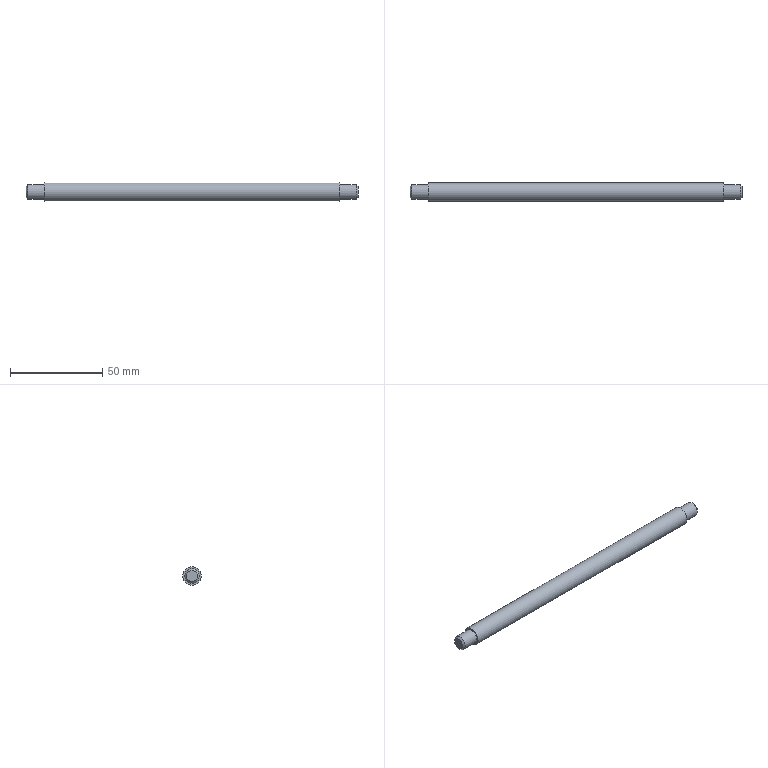Component | NX | HANDLE | 1 solid | 9 faces | box 180 x 10 x 10 mm | volume 13549 mm3 | plane 4 | cylinder 3 | cone 2 | commonest cylinder face diameters 8 x2 10 x1
STEP:
#1=CARTESIAN_POINT('',(0.,0.,0.));
#2=DIRECTION('',(0.,0.,1.));
#3=DIRECTION('',(1.,0.,0.));
#4=AXIS2_PLACEMENT_3D('',#1,#2,#3);
#5=CARTESIAN_POINT('',(80.,-135.,-189.));
#6=VERTEX_POINT('',#5);
#7=CARTESIAN_POINT('',(80.,-140.,-189.));
#8=DIRECTION('',(1.,0.,0.));
#9=DIRECTION('',(0.,1.,0.));
#10=AXIS2_PLACEMENT_3D('',#7,#8,#9);
#11=CIRCLE('',#10,5.);
#12=CARTESIAN_POINT('',(80.,-140.,-189.));
#13=DIRECTION('',(-1.,0.,0.));
#14=DIRECTION('',(0.,0.,1.));
#15=AXIS2_PLACEMENT_3D('',#12,#13,#14);
#16=CYLINDRICAL_SURFACE('',#15,5.);
#17=CARTESIAN_POINT('',(7.854,0.));
#18=DIRECTION('',(-1.,0.));
#19=VECTOR('',#18,1.);
#20=LINE('',#17,#19);
#21=(GEOMETRIC_REPRESENTATION_CONTEXT(2)PARAMETRIC_REPRESENTATION_CONTEXT()REPRESENTATION_CONTEXT('',''));
#22=DEFINITIONAL_REPRESENTATION('',(#20),#21);
#23=PCURVE('',#16,#22);
#24=CARTESIAN_POINT('',(80.,-140.,-189.));
#25=DIRECTION('',(1.,0.,0.));
#26=DIRECTION('',(0.,0.,-1.));
#27=AXIS2_PLACEMENT_3D('',#24,#25,#26);
#28=PLANE('',#27);
#29=CARTESIAN_POINT('',(0.,0.));
#30=DIRECTION('',(0.,1.));
#31=AXIS2_PLACEMENT_2D('',#29,#30);
#32=CIRCLE('',#31,5.);
#33=(GEOMETRIC_REPRESENTATION_CONTEXT(2)PARAMETRIC_REPRESENTATION_CONTEXT()REPRESENTATION_CONTEXT('',''));
#34=DEFINITIONAL_REPRESENTATION('',(#32),#33);
#35=PCURVE('',#28,#34);
#36=SURFACE_CURVE('',#11,(#23,#35),.PCURVE_S1.);
#37=EDGE_CURVE('',#6,#6,#36,.T.);
#38=ORIENTED_EDGE('',*,*,#37,.F.);
#39=CARTESIAN_POINT('',(-80.,-135.,-189.));
#40=VERTEX_POINT('',#39);
#41=CARTESIAN_POINT('',(80.,-135.,-189.));
#42=CARTESIAN_POINT('',(-80.,-135.,-189.));
#43=B_SPLINE_CURVE_WITH_KNOTS('',1,(#41,#42),.UNSPECIFIED.,.F.,.F.,(2,2),(0.,160.),.PIECEWISE_BEZIER_KNOTS.);
#44=CARTESIAN_POINT('',(7.854,0.));
#45=DIRECTION('',(0.,1.));
#46=VECTOR('',#45,1.);
#47=LINE('',#44,#46);
#48=(GEOMETRIC_REPRESENTATION_CONTEXT(2)PARAMETRIC_REPRESENTATION_CONTEXT()REPRESENTATION_CONTEXT('',''));
#49=DEFINITIONAL_REPRESENTATION('',(#47),#48);
#50=PCURVE('',#16,#49);
#51=CARTESIAN_POINT('',(1.571,0.));
#52=DIRECTION('',(0.,1.));
#53=VECTOR('',#52,1.);
#54=LINE('',#51,#53);
#55=(GEOMETRIC_REPRESENTATION_CONTEXT(2)PARAMETRIC_REPRESENTATION_CONTEXT()REPRESENTATION_CONTEXT('',''));
#56=DEFINITIONAL_REPRESENTATION('',(#54),#55);
#57=PCURVE('',#16,#56);
#58=SEAM_CURVE('',#43,(#50,#57),.PCURVE_S1.);
#59=EDGE_CURVE('',#6,#40,#58,.T.);
#60=ORIENTED_EDGE('',*,*,#59,.T.);
#61=CARTESIAN_POINT('',(-80.,-140.,-189.));
#62=DIRECTION('',(1.,0.,0.));
#63=DIRECTION('',(0.,1.,0.));
#64=AXIS2_PLACEMENT_3D('',#61,#62,#63);
#65=CIRCLE('',#64,5.);
#66=CARTESIAN_POINT('',(7.854,160.));
#67=DIRECTION('',(-1.,0.));
#68=VECTOR('',#67,1.);
#69=LINE('',#66,#68);
#70=(GEOMETRIC_REPRESENTATION_CONTEXT(2)PARAMETRIC_REPRESENTATION_CONTEXT()REPRESENTATION_CONTEXT('',''));
#71=DEFINITIONAL_REPRESENTATION('',(#69),#70);
#72=PCURVE('',#16,#71);
#73=CARTESIAN_POINT('',(-80.,-140.,-189.));
#74=DIRECTION('',(1.,0.,0.));
#75=DIRECTION('',(0.,0.,-1.));
#76=AXIS2_PLACEMENT_3D('',#73,#74,#75);
#77=PLANE('',#76);
#78=CARTESIAN_POINT('',(0.,0.));
#79=DIRECTION('',(0.,1.));
#80=AXIS2_PLACEMENT_2D('',#78,#79);
#81=CIRCLE('',#80,5.);
#82=(GEOMETRIC_REPRESENTATION_CONTEXT(2)PARAMETRIC_REPRESENTATION_CONTEXT()REPRESENTATION_CONTEXT('',''));
#83=DEFINITIONAL_REPRESENTATION('',(#81),#82);
#84=PCURVE('',#77,#83);
#85=SURFACE_CURVE('',#65,(#72,#84),.PCURVE_S1.);
#86=EDGE_CURVE('',#40,#40,#85,.T.);
#87=ORIENTED_EDGE('',*,*,#86,.T.);
#88=ORIENTED_EDGE('',*,*,#59,.F.);
#89=EDGE_LOOP('',(#38,#60,#87,#88));
#90=FACE_BOUND('',#89,.T.);
#91=ADVANCED_FACE('',(#90),#16,.T.);
#92=CARTESIAN_POINT('',(80.,-140.,-193.));
#93=VERTEX_POINT('',#92);
#94=CARTESIAN_POINT('',(80.,-140.,-189.));
#95=DIRECTION('',(-1.,0.,0.));
#96=DIRECTION('',(0.,0.,-1.));
#97=AXIS2_PLACEMENT_3D('',#94,#95,#96);
#98=CIRCLE('',#97,4.);
#99=CARTESIAN_POINT('',(4.,0.));
#100=CARTESIAN_POINT('',(4.,-6.928));
#101=CARTESIAN_POINT('',(-2.,-3.464));
#102=CARTESIAN_POINT('',(-8.,-0.));
#103=CARTESIAN_POINT('',(-2.,3.464));
#104=CARTESIAN_POINT('',(4.,6.928));
#105=CARTESIAN_POINT('',(4.,0.));
#106=(BOUNDED_CURVE()B_SPLINE_CURVE(2,(#99,#100,#101,#102,#103,#104,#105),.UNSPECIFIED.,.T.,.F.)B_SPLINE_CURVE_WITH_KNOTS((1,2,2,2,2,1),(-2.094,0.,2.094,4.189,6.283,8.378),.UNSPECIFIED.)CURVE()GEOMETRIC_REPRESENTATION_ITEM()RATIONAL_B_SPLINE_CURVE((1.,0.5,1.,0.5,1.,0.5,1.))REPRESENTATION_ITEM(''));
#107=(GEOMETRIC_REPRESENTATION_CONTEXT(2)PARAMETRIC_REPRESENTATION_CONTEXT()REPRESENTATION_CONTEXT('',''));
#108=DEFINITIONAL_REPRESENTATION('',(#106),#107);
#109=PCURVE('',#28,#108);
#110=CARTESIAN_POINT('',(90.,-140.,-189.));
#111=DIRECTION('',(-1.,0.,0.));
#112=DIRECTION('',(0.,0.,1.));
#113=AXIS2_PLACEMENT_3D('',#110,#111,#112);
#114=CYLINDRICAL_SURFACE('',#113,4.);
#115=CARTESIAN_POINT('',(3.142,10.));
#116=DIRECTION('',(1.,0.));
#117=VECTOR('',#116,1.);
#118=LINE('',#115,#117);
#119=(GEOMETRIC_REPRESENTATION_CONTEXT(2)PARAMETRIC_REPRESENTATION_CONTEXT()REPRESENTATION_CONTEXT('',''));
#120=DEFINITIONAL_REPRESENTATION('',(#118),#119);
#121=PCURVE('',#114,#120);
#122=SURFACE_CURVE('',#98,(#109,#121),.PCURVE_S1.);
#123=EDGE_CURVE('',#93,#93,#122,.T.);
#124=ORIENTED_EDGE('',*,*,#123,.T.);
#125=EDGE_LOOP('',(#124));
#126=FACE_BOUND('',#125,.T.);
#127=ORIENTED_EDGE('',*,*,#37,.T.);
#128=EDGE_LOOP('',(#127));
#129=FACE_BOUND('',#128,.T.);
#130=ADVANCED_FACE('',(#126,#129),#28,.T.);
#131=CARTESIAN_POINT('',(-80.,-140.,-193.));
#132=VERTEX_POINT('',#131);
#133=CARTESIAN_POINT('',(-80.,-140.,-189.));
#134=DIRECTION('',(-1.,0.,0.));
#135=DIRECTION('',(0.,0.,-1.));
#136=AXIS2_PLACEMENT_3D('',#133,#134,#135);
#137=CIRCLE('',#136,4.);
#138=CARTESIAN_POINT('',(4.,0.));
#139=CARTESIAN_POINT('',(4.,-6.928));
#140=CARTESIAN_POINT('',(-2.,-3.464));
#141=CARTESIAN_POINT('',(-8.,-0.));
#142=CARTESIAN_POINT('',(-2.,3.464));
#143=CARTESIAN_POINT('',(4.,6.928));
#144=CARTESIAN_POINT('',(4.,0.));
#145=(BOUNDED_CURVE()B_SPLINE_CURVE(2,(#138,#139,#140,#141,#142,#143,#144),.UNSPECIFIED.,.T.,.F.)B_SPLINE_CURVE_WITH_KNOTS((1,2,2,2,2,1),(-2.094,0.,2.094,4.189,6.283,8.378),.UNSPECIFIED.)CURVE()GEOMETRIC_REPRESENTATION_ITEM()RATIONAL_B_SPLINE_CURVE((1.,0.5,1.,0.5,1.,0.5,1.))REPRESENTATION_ITEM(''));
#146=(GEOMETRIC_REPRESENTATION_CONTEXT(2)PARAMETRIC_REPRESENTATION_CONTEXT()REPRESENTATION_CONTEXT('',''));
#147=DEFINITIONAL_REPRESENTATION('',(#145),#146);
#148=PCURVE('',#77,#147);
#149=CARTESIAN_POINT('',(90.,-140.,-189.));
#150=DIRECTION('',(-1.,0.,0.));
#151=DIRECTION('',(0.,0.,1.));
#152=AXIS2_PLACEMENT_3D('',#149,#150,#151);
#153=CYLINDRICAL_SURFACE('',#152,4.);
#154=CARTESIAN_POINT('',(3.142,170.));
#155=DIRECTION('',(1.,0.));
#156=VECTOR('',#155,1.);
#157=LINE('',#154,#156);
#158=(GEOMETRIC_REPRESENTATION_CONTEXT(2)PARAMETRIC_REPRESENTATION_CONTEXT()REPRESENTATION_CONTEXT('',''));
#159=DEFINITIONAL_REPRESENTATION('',(#157),#158);
#160=PCURVE('',#153,#159);
#161=SURFACE_CURVE('',#137,(#148,#160),.PCURVE_S1.);
#162=EDGE_CURVE('',#132,#132,#161,.T.);
#163=ORIENTED_EDGE('',*,*,#162,.F.);
#164=EDGE_LOOP('',(#163));
#165=FACE_BOUND('',#164,.T.);
#166=ORIENTED_EDGE('',*,*,#86,.F.);
#167=EDGE_LOOP('',(#166));
#168=FACE_BOUND('',#167,.T.);
#169=ADVANCED_FACE('',(#165,#168),#77,.F.);
#170=CARTESIAN_POINT('',(-90.,-140.,-192.));
#171=VERTEX_POINT('',#170);
#172=CARTESIAN_POINT('',(-90.,-140.,-189.));
#173=DIRECTION('',(-1.,0.,0.));
#174=DIRECTION('',(0.,0.,-1.));
#175=AXIS2_PLACEMENT_3D('',#172,#173,#174);
#176=CIRCLE('',#175,3.);
#177=CARTESIAN_POINT('',(-90.,-140.,-189.));
#178=DIRECTION('',(1.,0.,0.));
#179=DIRECTION('',(0.,0.,-1.));
#180=AXIS2_PLACEMENT_3D('',#177,#178,#179);
#181=PLANE('',#180);
#182=CARTESIAN_POINT('',(3.,0.));
#183=CARTESIAN_POINT('',(3.,-5.196));
#184=CARTESIAN_POINT('',(-1.5,-2.598));
#185=CARTESIAN_POINT('',(-6.,-0.));
#186=CARTESIAN_POINT('',(-1.5,2.598));
#187=CARTESIAN_POINT('',(3.,5.196));
#188=CARTESIAN_POINT('',(3.,0.));
#189=(BOUNDED_CURVE()B_SPLINE_CURVE(2,(#182,#183,#184,#185,#186,#187,#188),.UNSPECIFIED.,.T.,.F.)B_SPLINE_CURVE_WITH_KNOTS((1,2,2,2,2,1),(-2.094,0.,2.094,4.189,6.283,8.378),.UNSPECIFIED.)CURVE()GEOMETRIC_REPRESENTATION_ITEM()RATIONAL_B_SPLINE_CURVE((1.,0.5,1.,0.5,1.,0.5,1.))REPRESENTATION_ITEM(''));
#190=(GEOMETRIC_REPRESENTATION_CONTEXT(2)PARAMETRIC_REPRESENTATION_CONTEXT()REPRESENTATION_CONTEXT('',''));
#191=DEFINITIONAL_REPRESENTATION('',(#189),#190);
#192=PCURVE('',#181,#191);
#193=CARTESIAN_POINT('',(-89.,-140.,-189.));
#194=DIRECTION('',(1.,0.,0.));
#195=DIRECTION('',(0.,0.,-1.));
#196=AXIS2_PLACEMENT_3D('',#193,#194,#195);
#197=CONICAL_SURFACE('',#196,4.,0.7854);
#198=CARTESIAN_POINT('',(6.283,-1.));
#199=DIRECTION('',(-1.,0.));
#200=VECTOR('',#199,1.);
#201=LINE('',#198,#200);
#202=(GEOMETRIC_REPRESENTATION_CONTEXT(2)PARAMETRIC_REPRESENTATION_CONTEXT()REPRESENTATION_CONTEXT('',''));
#203=DEFINITIONAL_REPRESENTATION('',(#201),#202);
#204=PCURVE('',#197,#203);
#205=SURFACE_CURVE('',#176,(#192,#204),.PCURVE_S1.);
#206=EDGE_CURVE('',#171,#171,#205,.T.);
#207=ORIENTED_EDGE('',*,*,#206,.T.);
#208=EDGE_LOOP('',(#207));
#209=FACE_BOUND('',#208,.T.);
#210=ADVANCED_FACE('',(#209),#181,.F.);
#211=CARTESIAN_POINT('',(-89.,-140.,-193.));
#212=VERTEX_POINT('',#211);
#213=CARTESIAN_POINT('',(-89.,-140.,-189.));
#214=DIRECTION('',(1.,0.,0.));
#215=DIRECTION('',(0.,0.,-1.));
#216=AXIS2_PLACEMENT_3D('',#213,#214,#215);
#217=CIRCLE('',#216,4.);
#218=CARTESIAN_POINT('',(9.425,179.));
#219=DIRECTION('',(-1.,0.));
#220=VECTOR('',#219,1.);
#221=LINE('',#218,#220);
#222=(GEOMETRIC_REPRESENTATION_CONTEXT(2)PARAMETRIC_REPRESENTATION_CONTEXT()REPRESENTATION_CONTEXT('',''));
#223=DEFINITIONAL_REPRESENTATION('',(#221),#222);
#224=PCURVE('',#153,#223);
#225=CARTESIAN_POINT('',(0.,0.));
#226=DIRECTION('',(1.,0.));
#227=VECTOR('',#226,1.);
#228=LINE('',#225,#227);
#229=(GEOMETRIC_REPRESENTATION_CONTEXT(2)PARAMETRIC_REPRESENTATION_CONTEXT()REPRESENTATION_CONTEXT('',''));
#230=DEFINITIONAL_REPRESENTATION('',(#228),#229);
#231=PCURVE('',#197,#230);
#232=SURFACE_CURVE('',#217,(#224,#231),.PCURVE_S1.);
#233=EDGE_CURVE('',#212,#212,#232,.T.);
#234=ORIENTED_EDGE('',*,*,#233,.T.);
#235=CARTESIAN_POINT('',(-80.,-140.,-193.));
#236=CARTESIAN_POINT('',(-89.,-140.,-193.));
#237=B_SPLINE_CURVE_WITH_KNOTS('',1,(#235,#236),.UNSPECIFIED.,.F.,.F.,(2,2),(170.,179.),.PIECEWISE_BEZIER_KNOTS.);
#238=CARTESIAN_POINT('',(3.142,0.));
#239=DIRECTION('',(0.,1.));
#240=VECTOR('',#239,1.);
#241=LINE('',#238,#240);
#242=(GEOMETRIC_REPRESENTATION_CONTEXT(2)PARAMETRIC_REPRESENTATION_CONTEXT()REPRESENTATION_CONTEXT('',''));
#243=DEFINITIONAL_REPRESENTATION('',(#241),#242);
#244=PCURVE('',#153,#243);
#245=CARTESIAN_POINT('',(9.425,0.));
#246=DIRECTION('',(0.,1.));
#247=VECTOR('',#246,1.);
#248=LINE('',#245,#247);
#249=(GEOMETRIC_REPRESENTATION_CONTEXT(2)PARAMETRIC_REPRESENTATION_CONTEXT()REPRESENTATION_CONTEXT('',''));
#250=DEFINITIONAL_REPRESENTATION('',(#248),#249);
#251=PCURVE('',#153,#250);
#252=SEAM_CURVE('',#237,(#244,#251),.PCURVE_S1.);
#253=EDGE_CURVE('',#132,#212,#252,.T.);
#254=ORIENTED_EDGE('',*,*,#253,.F.);
#255=ORIENTED_EDGE('',*,*,#162,.T.);
#256=ORIENTED_EDGE('',*,*,#253,.T.);
#257=EDGE_LOOP('',(#234,#254,#255,#256));
#258=FACE_BOUND('',#257,.T.);
#259=ADVANCED_FACE('',(#258),#153,.T.);
#260=CARTESIAN_POINT('',(89.,-140.,-193.));
#261=VERTEX_POINT('',#260);
#262=CARTESIAN_POINT('',(89.,-140.,-189.));
#263=DIRECTION('',(-1.,0.,0.));
#264=DIRECTION('',(0.,0.,-1.));
#265=AXIS2_PLACEMENT_3D('',#262,#263,#264);
#266=CIRCLE('',#265,4.);
#267=CARTESIAN_POINT('',(3.142,1.));
#268=DIRECTION('',(1.,0.));
#269=VECTOR('',#268,1.);
#270=LINE('',#267,#269);
#271=(GEOMETRIC_REPRESENTATION_CONTEXT(2)PARAMETRIC_REPRESENTATION_CONTEXT()REPRESENTATION_CONTEXT('',''));
#272=DEFINITIONAL_REPRESENTATION('',(#270),#271);
#273=PCURVE('',#114,#272);
#274=CARTESIAN_POINT('',(90.,-140.,-189.));
#275=DIRECTION('',(-1.,0.,0.));
#276=DIRECTION('',(0.,0.,1.));
#277=AXIS2_PLACEMENT_3D('',#274,#275,#276);
#278=CONICAL_SURFACE('',#277,3.,0.7854);
#279=CARTESIAN_POINT('',(3.142,1.));
#280=DIRECTION('',(1.,0.));
#281=VECTOR('',#280,1.);
#282=LINE('',#279,#281);
#283=(GEOMETRIC_REPRESENTATION_CONTEXT(2)PARAMETRIC_REPRESENTATION_CONTEXT()REPRESENTATION_CONTEXT('',''));
#284=DEFINITIONAL_REPRESENTATION('',(#282),#283);
#285=PCURVE('',#278,#284);
#286=SURFACE_CURVE('',#266,(#273,#285),.PCURVE_S1.);
#287=EDGE_CURVE('',#261,#261,#286,.T.);
#288=ORIENTED_EDGE('',*,*,#287,.T.);
#289=CARTESIAN_POINT('',(89.,-140.,-193.));
#290=CARTESIAN_POINT('',(80.,-140.,-193.));
#291=B_SPLINE_CURVE_WITH_KNOTS('',1,(#289,#290),.UNSPECIFIED.,.F.,.F.,(2,2),(1.,10.),.PIECEWISE_BEZIER_KNOTS.);
#292=CARTESIAN_POINT('',(9.425,0.));
#293=DIRECTION('',(0.,1.));
#294=VECTOR('',#293,1.);
#295=LINE('',#292,#294);
#296=(GEOMETRIC_REPRESENTATION_CONTEXT(2)PARAMETRIC_REPRESENTATION_CONTEXT()REPRESENTATION_CONTEXT('',''));
#297=DEFINITIONAL_REPRESENTATION('',(#295),#296);
#298=PCURVE('',#114,#297);
#299=CARTESIAN_POINT('',(3.142,0.));
#300=DIRECTION('',(0.,1.));
#301=VECTOR('',#300,1.);
#302=LINE('',#299,#301);
#303=(GEOMETRIC_REPRESENTATION_CONTEXT(2)PARAMETRIC_REPRESENTATION_CONTEXT()REPRESENTATION_CONTEXT('',''));
#304=DEFINITIONAL_REPRESENTATION('',(#302),#303);
#305=PCURVE('',#114,#304);
#306=SEAM_CURVE('',#291,(#298,#305),.PCURVE_S1.);
#307=EDGE_CURVE('',#261,#93,#306,.T.);
#308=ORIENTED_EDGE('',*,*,#307,.T.);
#309=ORIENTED_EDGE('',*,*,#123,.F.);
#310=ORIENTED_EDGE('',*,*,#307,.F.);
#311=EDGE_LOOP('',(#288,#308,#309,#310));
#312=FACE_BOUND('',#311,.T.);
#313=ADVANCED_FACE('',(#312),#114,.T.);
#314=CARTESIAN_POINT('',(90.,-140.,-192.));
#315=VERTEX_POINT('',#314);
#316=CARTESIAN_POINT('',(90.,-140.,-189.));
#317=DIRECTION('',(1.,0.,0.));
#318=DIRECTION('',(0.,0.,-1.));
#319=AXIS2_PLACEMENT_3D('',#316,#317,#318);
#320=CIRCLE('',#319,3.);
#321=CARTESIAN_POINT('',(90.,-140.,-189.));
#322=DIRECTION('',(1.,0.,0.));
#323=DIRECTION('',(0.,0.,-1.));
#324=AXIS2_PLACEMENT_3D('',#321,#322,#323);
#325=PLANE('',#324);
#326=CARTESIAN_POINT('',(0.,0.));
#327=DIRECTION('',(1.,0.));
#328=AXIS2_PLACEMENT_2D('',#326,#327);
#329=CIRCLE('',#328,3.);
#330=(GEOMETRIC_REPRESENTATION_CONTEXT(2)PARAMETRIC_REPRESENTATION_CONTEXT()REPRESENTATION_CONTEXT('',''));
#331=DEFINITIONAL_REPRESENTATION('',(#329),#330);
#332=PCURVE('',#325,#331);
#333=CARTESIAN_POINT('',(9.425,0.));
#334=DIRECTION('',(-1.,0.));
#335=VECTOR('',#334,1.);
#336=LINE('',#333,#335);
#337=(GEOMETRIC_REPRESENTATION_CONTEXT(2)PARAMETRIC_REPRESENTATION_CONTEXT()REPRESENTATION_CONTEXT('',''));
#338=DEFINITIONAL_REPRESENTATION('',(#336),#337);
#339=PCURVE('',#278,#338);
#340=SURFACE_CURVE('',#320,(#332,#339),.PCURVE_S1.);
#341=EDGE_CURVE('',#315,#315,#340,.T.);
#342=ORIENTED_EDGE('',*,*,#341,.T.);
#343=EDGE_LOOP('',(#342));
#344=FACE_BOUND('',#343,.T.);
#345=ADVANCED_FACE('',(#344),#325,.T.);
#346=ORIENTED_EDGE('',*,*,#206,.F.);
#347=CARTESIAN_POINT('',(-90.,-140.,-192.));
#348=CARTESIAN_POINT('',(-89.,-140.,-193.));
#349=B_SPLINE_CURVE_WITH_KNOTS('',1,(#347,#348),.UNSPECIFIED.,.F.,.F.,(2,2),(-1.414,0.),.PIECEWISE_BEZIER_KNOTS.);
#350=CARTESIAN_POINT('',(6.283,0.));
#351=DIRECTION('',(0.,1.));
#352=VECTOR('',#351,1.);
#353=LINE('',#350,#352);
#354=(GEOMETRIC_REPRESENTATION_CONTEXT(2)PARAMETRIC_REPRESENTATION_CONTEXT()REPRESENTATION_CONTEXT('',''));
#355=DEFINITIONAL_REPRESENTATION('',(#353),#354);
#356=PCURVE('',#197,#355);
#357=CARTESIAN_POINT('',(0.,0.));
#358=DIRECTION('',(0.,1.));
#359=VECTOR('',#358,1.);
#360=LINE('',#357,#359);
#361=(GEOMETRIC_REPRESENTATION_CONTEXT(2)PARAMETRIC_REPRESENTATION_CONTEXT()REPRESENTATION_CONTEXT('',''));
#362=DEFINITIONAL_REPRESENTATION('',(#360),#361);
#363=PCURVE('',#197,#362);
#364=SEAM_CURVE('',#349,(#356,#363),.PCURVE_S1.);
#365=EDGE_CURVE('',#171,#212,#364,.T.);
#366=ORIENTED_EDGE('',*,*,#365,.T.);
#367=ORIENTED_EDGE('',*,*,#233,.F.);
#368=ORIENTED_EDGE('',*,*,#365,.F.);
#369=EDGE_LOOP('',(#346,#366,#367,#368));
#370=FACE_BOUND('',#369,.T.);
#371=ADVANCED_FACE('',(#370),#197,.T.);
#372=ORIENTED_EDGE('',*,*,#287,.F.);
#373=CARTESIAN_POINT('',(90.,-140.,-192.));
#374=CARTESIAN_POINT('',(89.,-140.,-193.));
#375=B_SPLINE_CURVE_WITH_KNOTS('',1,(#373,#374),.UNSPECIFIED.,.F.,.F.,(2,2),(0.,1.414),.PIECEWISE_BEZIER_KNOTS.);
#376=CARTESIAN_POINT('',(3.142,0.));
#377=DIRECTION('',(0.,1.));
#378=VECTOR('',#377,1.);
#379=LINE('',#376,#378);
#380=(GEOMETRIC_REPRESENTATION_CONTEXT(2)PARAMETRIC_REPRESENTATION_CONTEXT()REPRESENTATION_CONTEXT('',''));
#381=DEFINITIONAL_REPRESENTATION('',(#379),#380);
#382=PCURVE('',#278,#381);
#383=CARTESIAN_POINT('',(9.425,0.));
#384=DIRECTION('',(0.,1.));
#385=VECTOR('',#384,1.);
#386=LINE('',#383,#385);
#387=(GEOMETRIC_REPRESENTATION_CONTEXT(2)PARAMETRIC_REPRESENTATION_CONTEXT()REPRESENTATION_CONTEXT('',''));
#388=DEFINITIONAL_REPRESENTATION('',(#386),#387);
#389=PCURVE('',#278,#388);
#390=SEAM_CURVE('',#375,(#382,#389),.PCURVE_S1.);
#391=EDGE_CURVE('',#315,#261,#390,.T.);
#392=ORIENTED_EDGE('',*,*,#391,.F.);
#393=ORIENTED_EDGE('',*,*,#341,.F.);
#394=ORIENTED_EDGE('',*,*,#391,.T.);
#395=EDGE_LOOP('',(#372,#392,#393,#394));
#396=FACE_BOUND('',#395,.T.);
#397=ADVANCED_FACE('',(#396),#278,.T.);
#398=CLOSED_SHELL('',(#91,#130,#169,#210,#259,#313,#345,#371,#397));
#399=MANIFOLD_SOLID_BREP('',#398);
#400=(LENGTH_UNIT()NAMED_UNIT(*)SI_UNIT(.MILLI.,.METRE.));
#401=UNCERTAINTY_MEASURE_WITH_UNIT(LENGTH_MEASURE(0.00001),#400,'','');
#402=(NAMED_UNIT(*)PLANE_ANGLE_UNIT()SI_UNIT($,.RADIAN.));
#403=(NAMED_UNIT(*)SI_UNIT($,.STERADIAN.)SOLID_ANGLE_UNIT());
#404=(GEOMETRIC_REPRESENTATION_CONTEXT(3)GLOBAL_UNCERTAINTY_ASSIGNED_CONTEXT((#401))GLOBAL_UNIT_ASSIGNED_CONTEXT((#400,#402,#403))REPRESENTATION_CONTEXT('',''));
#405=ADVANCED_BREP_SHAPE_REPRESENTATION('',(#4,#399),#404);